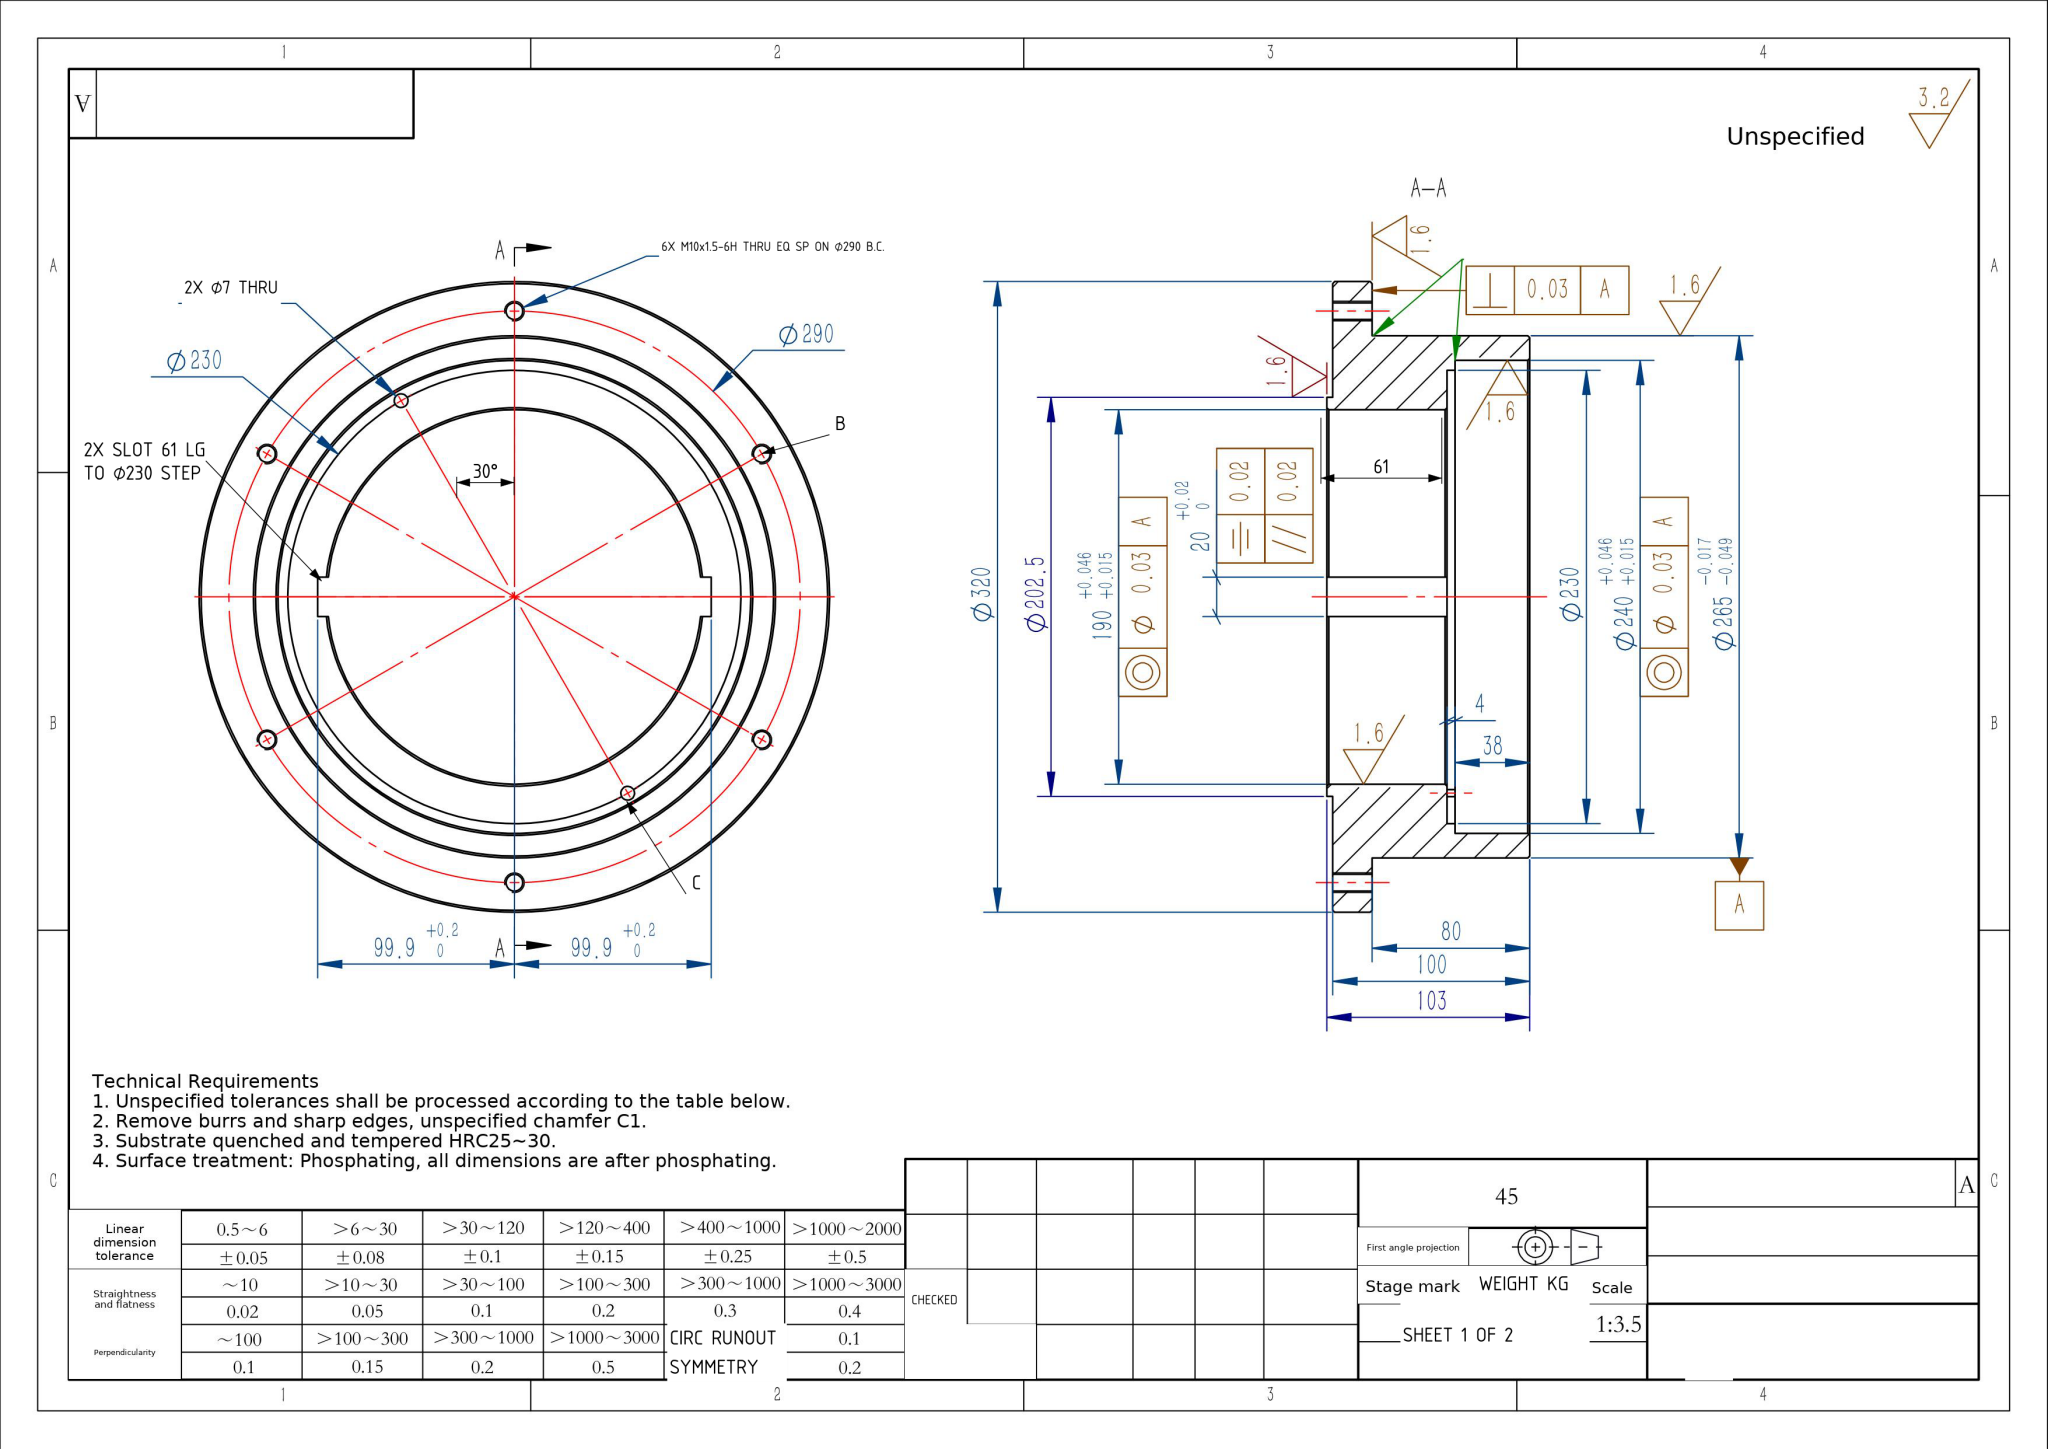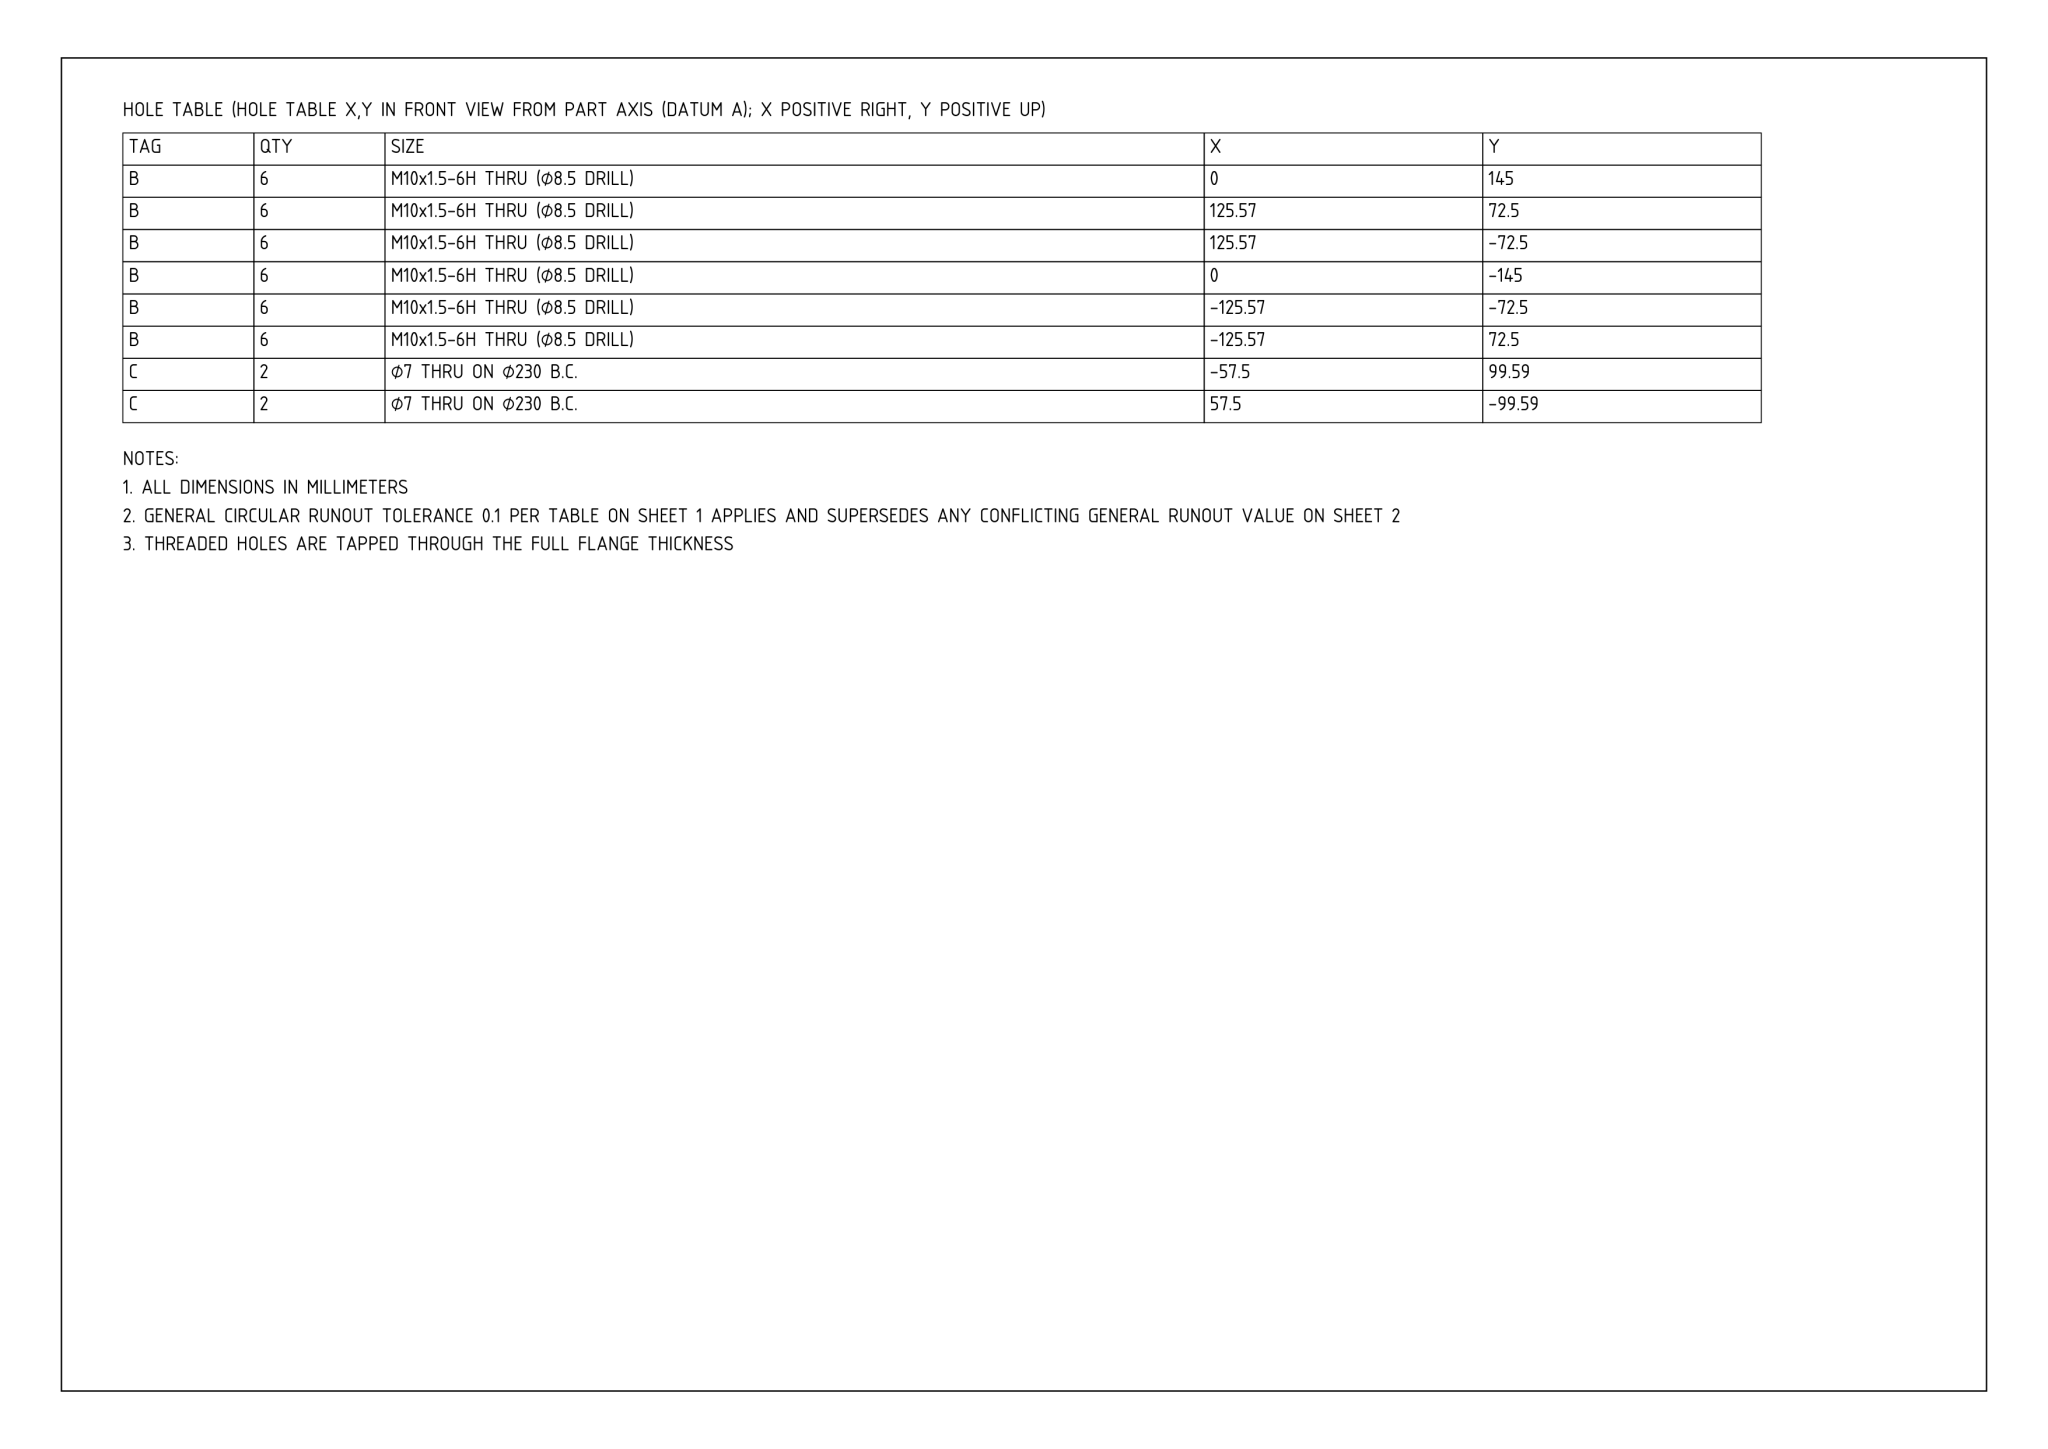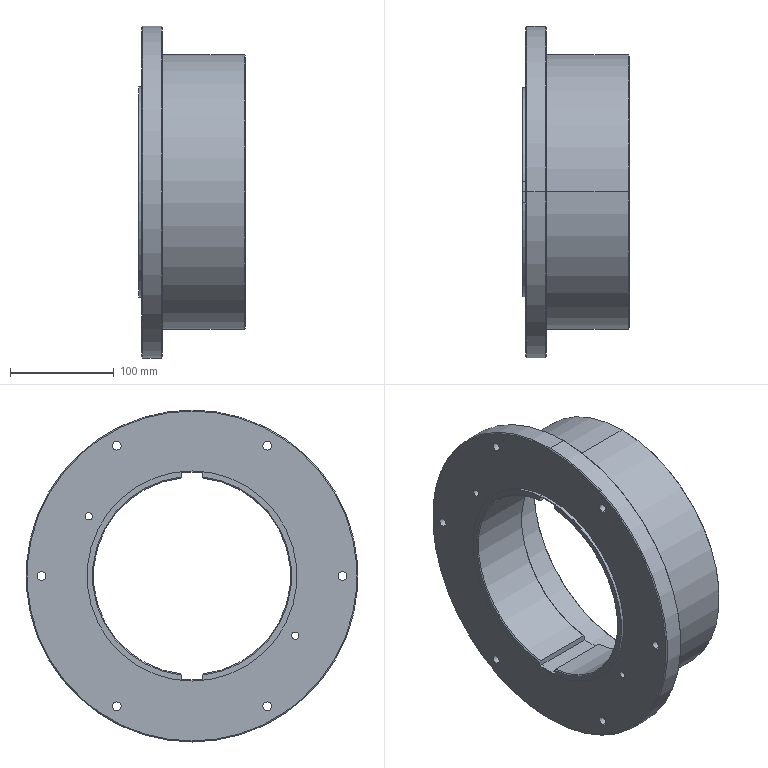Part | NX | mm | 1 solid | 53 faces | box 103 x 320 x 320 mm | volume 2476517 mm3 | cylinder 29 | cone 12 | plane 12 | commonest cylinder face diameters 8.5 x12 7 x4 230 x3 320 x2 265 x2 240 x2 202.5 x2 190 x2